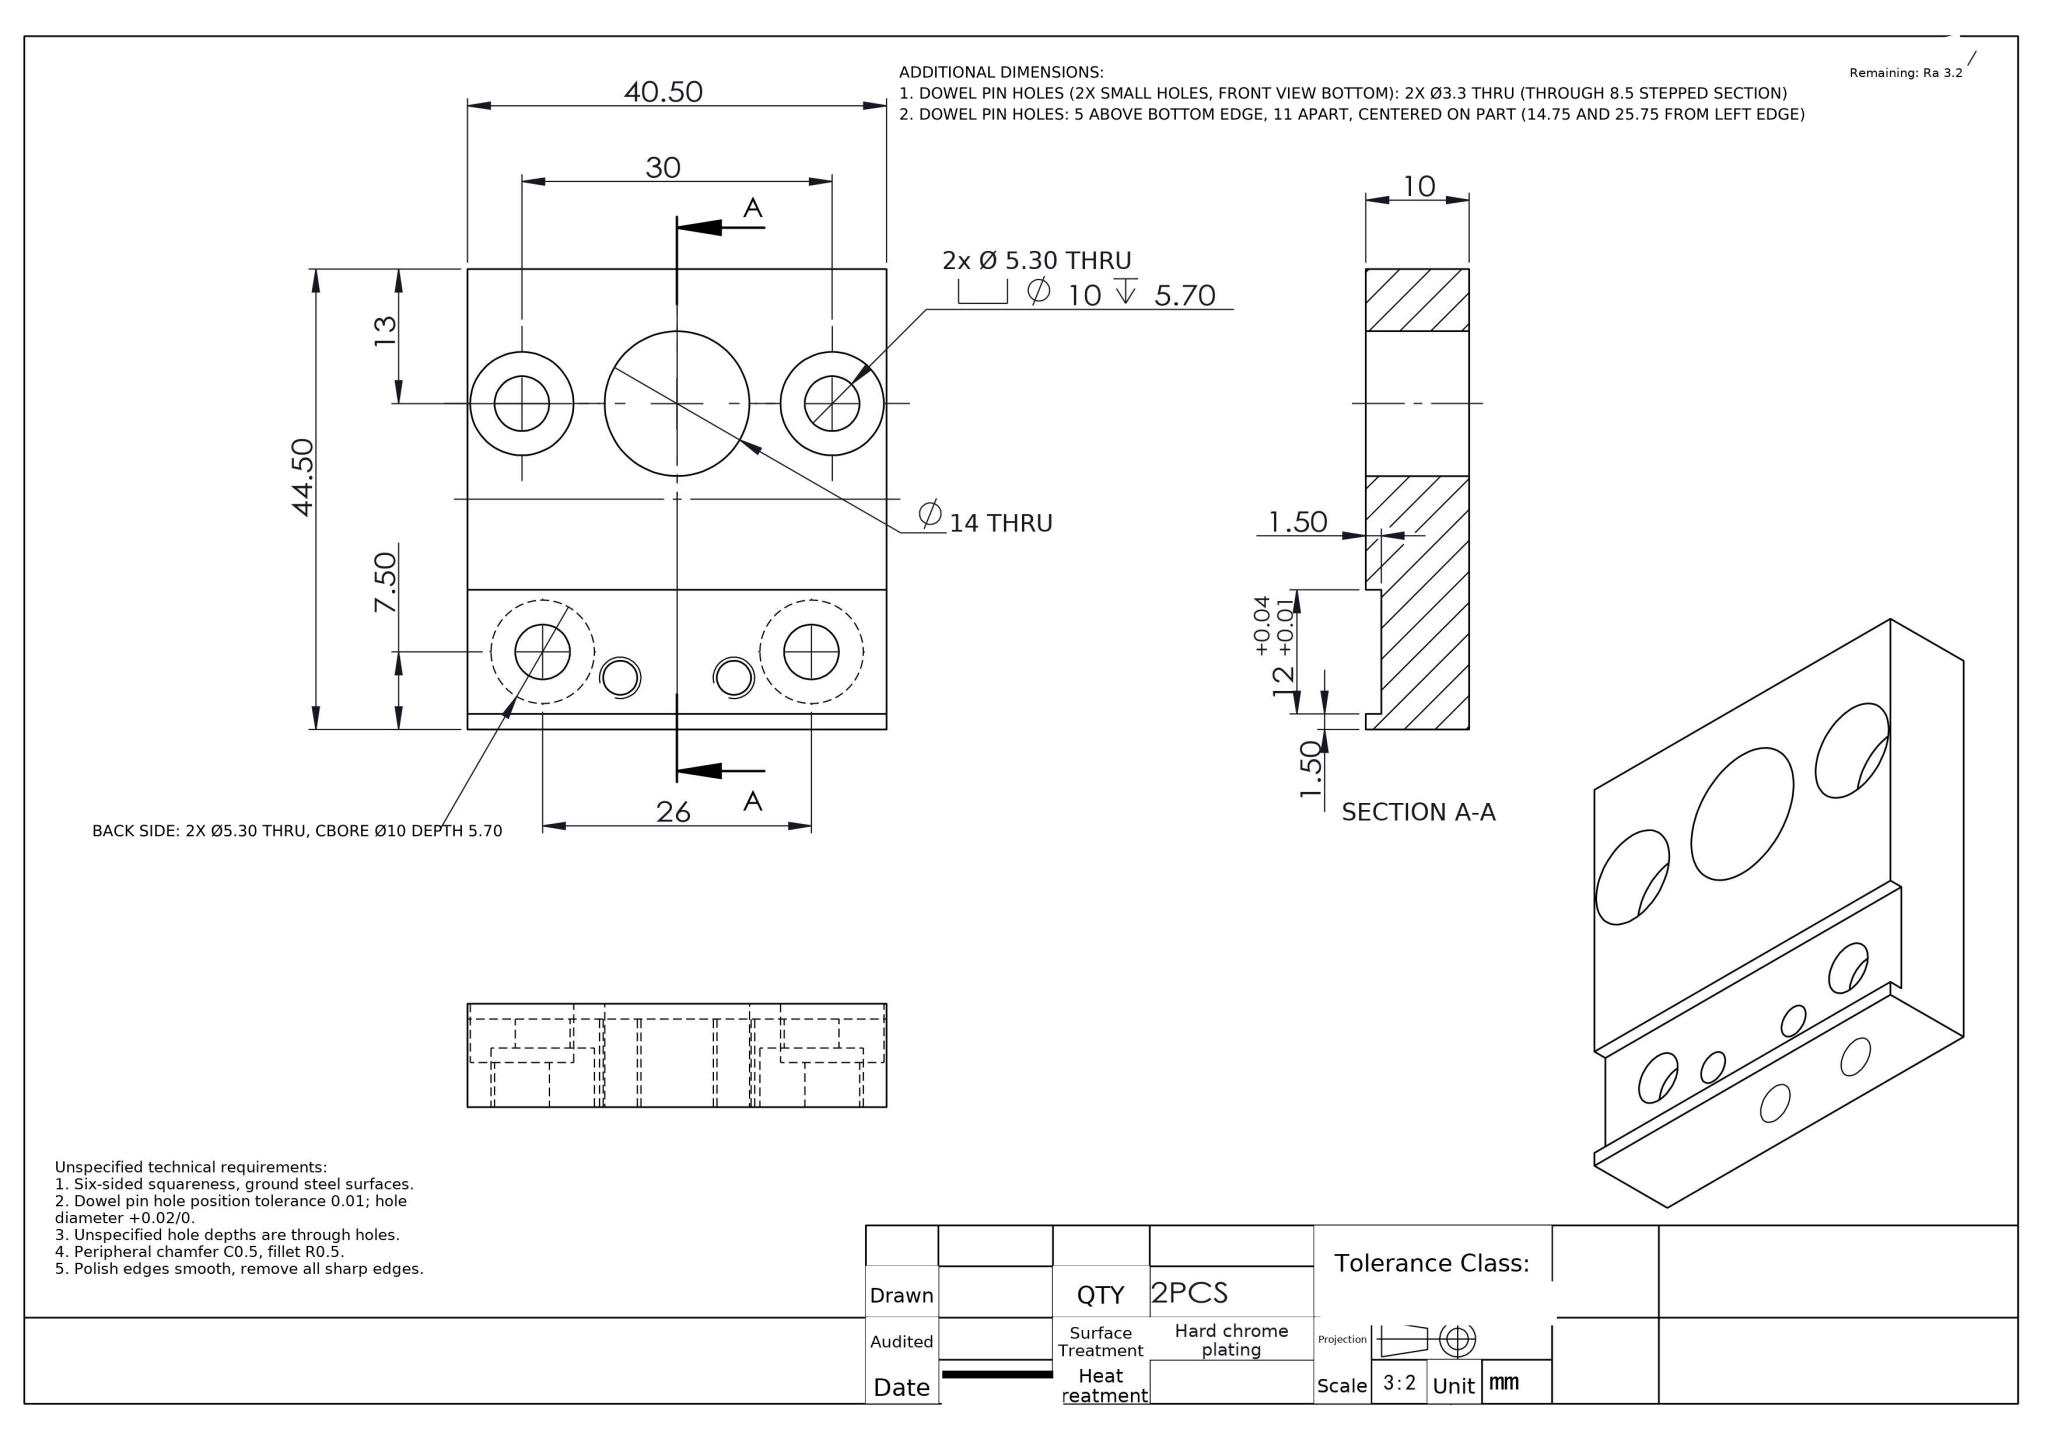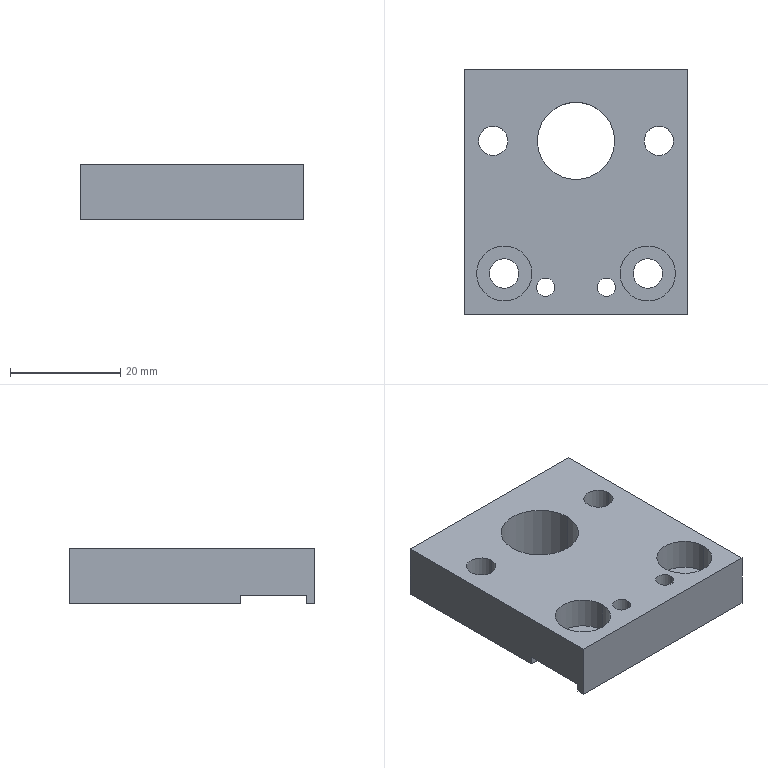Part | NX | mm | 1 solid | 36 faces | box 40.5 x 44.5 x 10 mm | volume 13505 mm3 | cylinder 22 | plane 14 | commonest cylinder face diameters 10 x8 5.3 x8 3.3 x4 14 x2